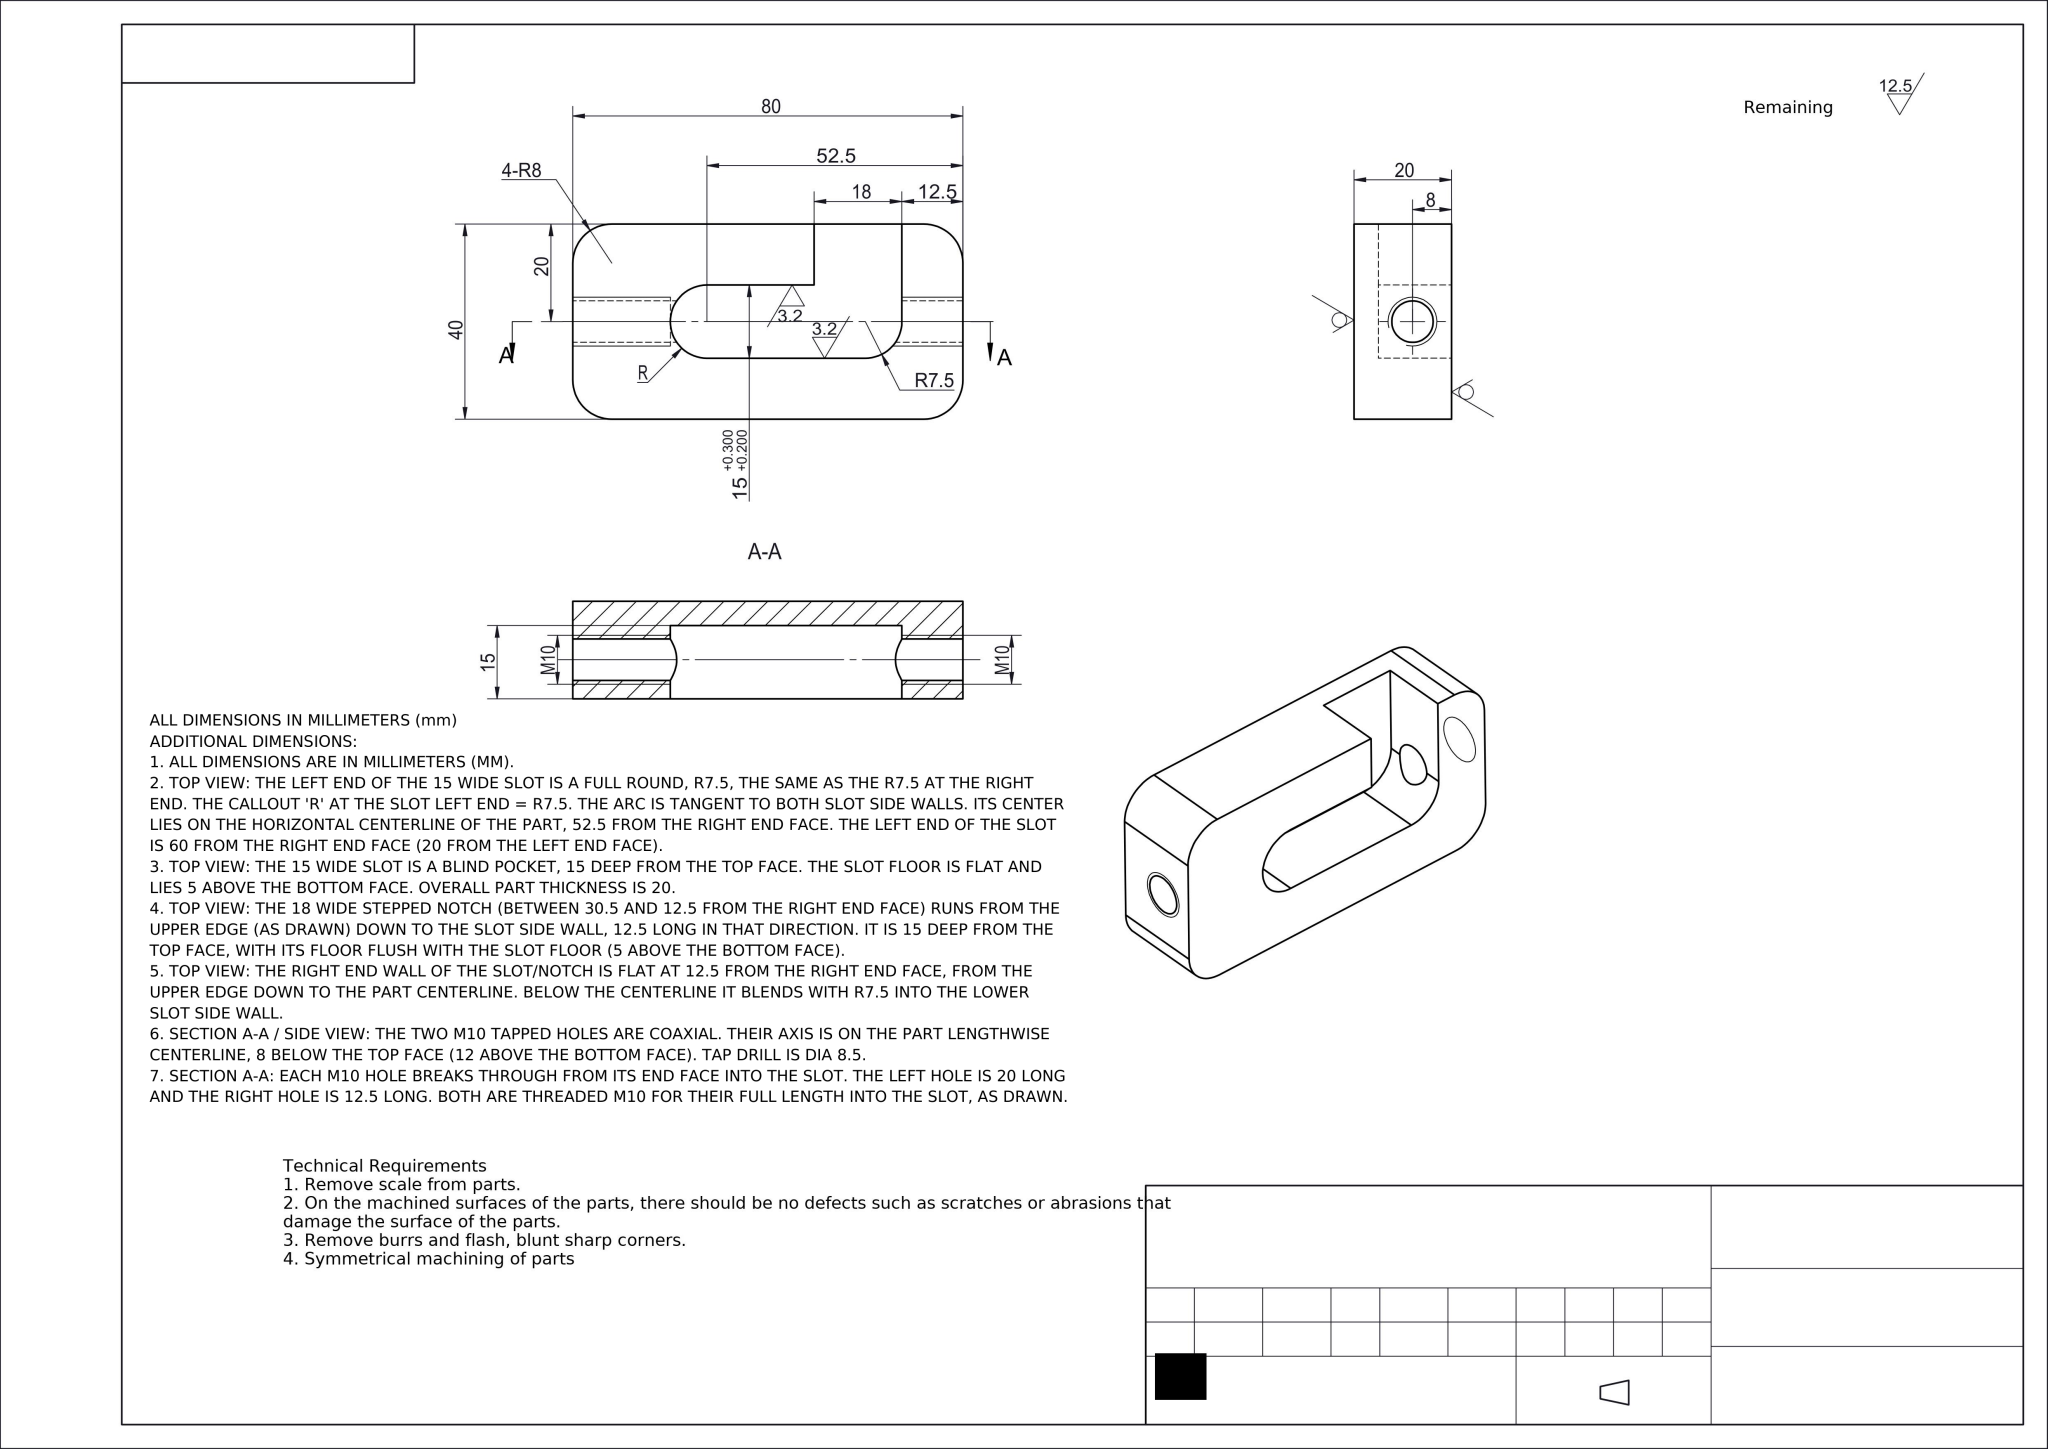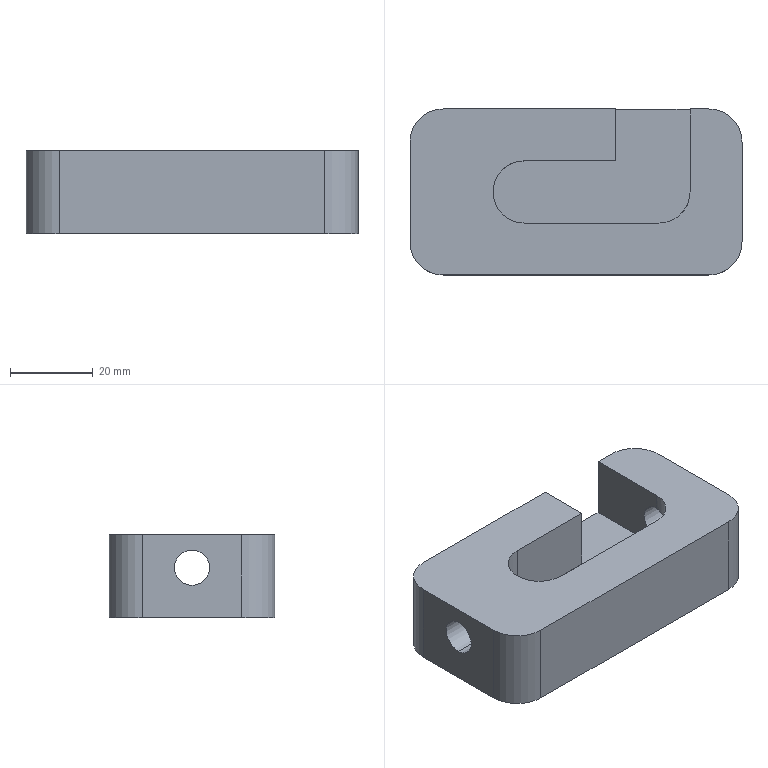Part | NX | mm | U-Shaped Slotted Clevis Bracket | 1 solid | 21 faces | box 80 x 40 x 20 mm | volume 47511 mm3 | plane 11 | cylinder 10 | commonest cylinder face diameters 8.5 x4 16 x4 15 x2
STEP:
#1=COLOUR_RGB('',1.,1.,1.);
#2=FILL_AREA_STYLE_COLOUR('',#1);
#3=FILL_AREA_STYLE('',(#2));
#4=SURFACE_STYLE_FILL_AREA(#3);
#5=SURFACE_SIDE_STYLE('',(#4));
#6=SURFACE_STYLE_USAGE(.BOTH.,#5);
#7=PRESENTATION_STYLE_ASSIGNMENT((#6));
#8=CARTESIAN_POINT('',(27.5,0.,16.25));
#9=VERTEX_POINT('',#8);
#10=CARTESIAN_POINT('',(27.5,0.,7.75));
#11=VERTEX_POINT('',#10);
#12=CARTESIAN_POINT('',(27.5,0.,16.25));
#13=CARTESIAN_POINT('',(27.5,-0.2876,16.25));
#14=CARTESIAN_POINT('',(27.484,-0.5693,16.221));
#15=CARTESIAN_POINT('',(27.421,-1.122,16.109));
#16=CARTESIAN_POINT('',(27.374,-1.395,16.024));
#17=CARTESIAN_POINT('',(27.258,-1.908,15.808));
#18=CARTESIAN_POINT('',(27.189,-2.15,15.676));
#19=CARTESIAN_POINT('',(27.036,-2.607,15.367));
#20=CARTESIAN_POINT('',(26.954,-2.818,15.193));
#21=CARTESIAN_POINT('',(26.786,-3.201,14.809));
#22=CARTESIAN_POINT('',(26.7,-3.376,14.597));
#23=CARTESIAN_POINT('',(26.537,-3.68,14.143));
#24=CARTESIAN_POINT('',(26.462,-3.81,13.904));
#25=CARTESIAN_POINT('',(26.331,-4.024,13.396));
#26=CARTESIAN_POINT('',(26.275,-4.108,13.124));
#27=CARTESIAN_POINT('',(26.2,-4.221,12.571));
#28=CARTESIAN_POINT('',(26.18,-4.25,12.289));
#29=CARTESIAN_POINT('',(26.18,-4.25,11.714));
#30=CARTESIAN_POINT('',(26.2,-4.221,11.432));
#31=CARTESIAN_POINT('',(26.274,-4.109,10.879));
#32=CARTESIAN_POINT('',(26.33,-4.025,10.607));
#33=CARTESIAN_POINT('',(26.461,-3.81,10.097));
#34=CARTESIAN_POINT('',(26.538,-3.678,9.854));
#35=CARTESIAN_POINT('',(26.701,-3.372,9.399));
#36=CARTESIAN_POINT('',(26.786,-3.2,9.19));
#37=CARTESIAN_POINT('',(26.955,-2.816,8.805));
#38=CARTESIAN_POINT('',(27.038,-2.602,8.628));
#39=CARTESIAN_POINT('',(27.19,-2.149,8.323));
#40=CARTESIAN_POINT('',(27.258,-1.908,8.192));
#41=CARTESIAN_POINT('',(27.345,-1.522,8.029));
#42=CARTESIAN_POINT('',(27.372,-1.389,7.981));
#43=CARTESIAN_POINT('',(27.417,-1.119,7.898));
#44=CARTESIAN_POINT('',(27.437,-0.9829,7.863));
#45=CARTESIAN_POINT('',(27.483,-0.5695,7.779));
#46=CARTESIAN_POINT('',(27.5,-0.288,7.75));
#47=CARTESIAN_POINT('',(27.5,0.,7.75));
#48=B_SPLINE_CURVE_WITH_KNOTS('',3,(#12,#13,#14,#15,#16,#17,#18,#19,#20,#21,#22,#23,#24,#25,#26,#27,#28,#29,#30,#31,#32,#33,#34,#35,#36,#37,#38,#39,#40,#41,#42,#43,#44,#45,#46,#47),.UNSPECIFIED.,.F.,.F.,(4,2,2,2,2,2,2,2,2,2,2,2,2,2,2,2,2,4),(0.,0.0008494,0.001699,0.002548,0.003398,0.004247,0.005097,0.005946,0.006796,0.007645,0.008494,0.009344,0.01019,0.01104,0.01189,0.01232,0.01274,0.01359),.UNSPECIFIED.);
#49=EDGE_CURVE('',#9,#11,#48,.T.);
#50=ORIENTED_EDGE('',*,*,#49,.F.);
#51=CARTESIAN_POINT('',(40.,-0.,16.25));
#52=VERTEX_POINT('',#51);
#53=CARTESIAN_POINT('',(40.,-0.,16.25));
#54=DIRECTION('',(1.,-0.,0.));
#55=VECTOR('',#54,1000.);
#56=LINE('',#53,#55);
#57=EDGE_CURVE('',#9,#52,#56,.T.);
#58=ORIENTED_EDGE('',*,*,#57,.T.);
#59=CARTESIAN_POINT('',(40.,-0.,7.75));
#60=VERTEX_POINT('',#59);
#61=CARTESIAN_POINT('',(40.,-0.,12.));
#62=DIRECTION('',(1.,-0.,0.));
#63=DIRECTION('',(0.,0.,-1.));
#64=AXIS2_PLACEMENT_3D('',#61,#62,#63);
#65=CIRCLE('',#64,4.25);
#66=EDGE_CURVE('',#52,#60,#65,.T.);
#67=ORIENTED_EDGE('',*,*,#66,.T.);
#68=CARTESIAN_POINT('',(40.,-0.,7.75));
#69=DIRECTION('',(1.,-0.,0.));
#70=VECTOR('',#69,1000.);
#71=LINE('',#68,#70);
#72=EDGE_CURVE('',#11,#60,#71,.T.);
#73=ORIENTED_EDGE('',*,*,#72,.F.);
#74=EDGE_LOOP('',(#50,#58,#67,#73));
#75=FACE_OUTER_BOUND('',#74,.T.);
#76=CARTESIAN_POINT('',(40.,-0.,12.));
#77=DIRECTION('',(1.,-0.,0.));
#78=DIRECTION('',(0.,0.,-1.));
#79=AXIS2_PLACEMENT_3D('',#76,#77,#78);
#80=CYLINDRICAL_SURFACE('',#79,4.25);
#81=ADVANCED_FACE('',(#75),#80,.F.);
#82=CARTESIAN_POINT('',(-20.,0.,7.75));
#83=VERTEX_POINT('',#82);
#84=CARTESIAN_POINT('',(-20.,0.,16.25));
#85=VERTEX_POINT('',#84);
#86=CARTESIAN_POINT('',(-20.,0.,7.75));
#87=CARTESIAN_POINT('',(-20.,-0.2872,7.75));
#88=CARTESIAN_POINT('',(-19.984,-0.5694,7.779));
#89=CARTESIAN_POINT('',(-19.921,-1.122,7.891));
#90=CARTESIAN_POINT('',(-19.874,-1.395,7.976));
#91=CARTESIAN_POINT('',(-19.758,-1.908,8.192));
#92=CARTESIAN_POINT('',(-19.689,-2.15,8.324));
#93=CARTESIAN_POINT('',(-19.536,-2.608,8.633));
#94=CARTESIAN_POINT('',(-19.454,-2.818,8.807));
#95=CARTESIAN_POINT('',(-19.286,-3.201,9.191));
#96=CARTESIAN_POINT('',(-19.2,-3.375,9.403));
#97=CARTESIAN_POINT('',(-19.038,-3.679,9.856));
#98=CARTESIAN_POINT('',(-18.962,-3.809,10.095));
#99=CARTESIAN_POINT('',(-18.831,-4.023,10.603));
#100=CARTESIAN_POINT('',(-18.775,-4.108,10.875));
#101=CARTESIAN_POINT('',(-18.7,-4.221,11.426));
#102=CARTESIAN_POINT('',(-18.68,-4.25,11.71));
#103=CARTESIAN_POINT('',(-18.679,-4.25,12.284));
#104=CARTESIAN_POINT('',(-18.699,-4.222,12.565));
#105=CARTESIAN_POINT('',(-18.774,-4.11,13.118));
#106=CARTESIAN_POINT('',(-18.829,-4.026,13.39));
#107=CARTESIAN_POINT('',(-18.96,-3.812,13.9));
#108=CARTESIAN_POINT('',(-19.038,-3.68,14.144));
#109=CARTESIAN_POINT('',(-19.2,-3.374,14.598));
#110=CARTESIAN_POINT('',(-19.285,-3.202,14.807));
#111=CARTESIAN_POINT('',(-19.453,-2.818,15.193));
#112=CARTESIAN_POINT('',(-19.537,-2.605,15.369));
#113=CARTESIAN_POINT('',(-19.688,-2.153,15.674));
#114=CARTESIAN_POINT('',(-19.757,-1.912,15.806));
#115=CARTESIAN_POINT('',(-19.873,-1.398,16.023));
#116=CARTESIAN_POINT('',(-19.92,-1.126,16.108));
#117=CARTESIAN_POINT('',(-19.983,-0.5735,16.221));
#118=CARTESIAN_POINT('',(-20.,-0.287,16.25));
#119=CARTESIAN_POINT('',(-20.,0.,16.25));
#120=B_SPLINE_CURVE_WITH_KNOTS('',3,(#86,#87,#88,#89,#90,#91,#92,#93,#94,#95,#96,#97,#98,#99,#100,#101,#102,#103,#104,#105,#106,#107,#108,#109,#110,#111,#112,#113,#114,#115,#116,#117,#118,#119),.UNSPECIFIED.,.F.,.F.,(4,2,2,2,2,2,2,2,2,2,2,2,2,2,2,2,4),(0.01359,0.01444,0.01529,0.01613,0.01698,0.01783,0.01868,0.01953,0.02037,0.02122,0.02207,0.02292,0.02376,0.02461,0.02546,0.02631,0.02716),.UNSPECIFIED.);
#121=EDGE_CURVE('',#83,#85,#120,.T.);
#122=ORIENTED_EDGE('',*,*,#121,.F.);
#123=CARTESIAN_POINT('',(-40.,0.,7.75));
#124=VERTEX_POINT('',#123);
#125=CARTESIAN_POINT('',(-40.,0.,7.75));
#126=DIRECTION('',(-1.,0.,-0.));
#127=VECTOR('',#126,1000.);
#128=LINE('',#125,#127);
#129=EDGE_CURVE('',#83,#124,#128,.T.);
#130=ORIENTED_EDGE('',*,*,#129,.T.);
#131=CARTESIAN_POINT('',(-40.,0.,16.25));
#132=VERTEX_POINT('',#131);
#133=CARTESIAN_POINT('',(-40.,0.,12.));
#134=DIRECTION('',(-1.,0.,-0.));
#135=DIRECTION('',(0.,0.,1.));
#136=AXIS2_PLACEMENT_3D('',#133,#134,#135);
#137=CIRCLE('',#136,4.25);
#138=EDGE_CURVE('',#124,#132,#137,.T.);
#139=ORIENTED_EDGE('',*,*,#138,.T.);
#140=CARTESIAN_POINT('',(-40.,0.,16.25));
#141=DIRECTION('',(-1.,0.,-0.));
#142=VECTOR('',#141,1000.);
#143=LINE('',#140,#142);
#144=EDGE_CURVE('',#85,#132,#143,.T.);
#145=ORIENTED_EDGE('',*,*,#144,.F.);
#146=EDGE_LOOP('',(#122,#130,#139,#145));
#147=FACE_OUTER_BOUND('',#146,.T.);
#148=CARTESIAN_POINT('',(-40.,0.,12.));
#149=DIRECTION('',(-1.,0.,-0.));
#150=DIRECTION('',(0.,0.,1.));
#151=AXIS2_PLACEMENT_3D('',#148,#149,#150);
#152=CYLINDRICAL_SURFACE('',#151,4.25);
#153=ADVANCED_FACE('',(#147),#152,.F.);
#154=CARTESIAN_POINT('',(-20.,0.,16.25));
#155=CARTESIAN_POINT('',(-20.,0.2876,16.25));
#156=CARTESIAN_POINT('',(-19.984,0.5693,16.221));
#157=CARTESIAN_POINT('',(-19.921,1.122,16.109));
#158=CARTESIAN_POINT('',(-19.874,1.395,16.024));
#159=CARTESIAN_POINT('',(-19.758,1.908,15.808));
#160=CARTESIAN_POINT('',(-19.689,2.15,15.676));
#161=CARTESIAN_POINT('',(-19.536,2.608,15.367));
#162=CARTESIAN_POINT('',(-19.454,2.818,15.193));
#163=CARTESIAN_POINT('',(-19.286,3.201,14.809));
#164=CARTESIAN_POINT('',(-19.2,3.376,14.596));
#165=CARTESIAN_POINT('',(-19.037,3.68,14.143));
#166=CARTESIAN_POINT('',(-18.961,3.81,13.903));
#167=CARTESIAN_POINT('',(-18.83,4.024,13.396));
#168=CARTESIAN_POINT('',(-18.775,4.108,13.124));
#169=CARTESIAN_POINT('',(-18.7,4.221,12.571));
#170=CARTESIAN_POINT('',(-18.68,4.25,12.289));
#171=CARTESIAN_POINT('',(-18.68,4.25,11.713));
#172=CARTESIAN_POINT('',(-18.7,4.221,11.432));
#173=CARTESIAN_POINT('',(-18.774,4.109,10.879));
#174=CARTESIAN_POINT('',(-18.83,4.025,10.607));
#175=CARTESIAN_POINT('',(-18.961,3.81,10.097));
#176=CARTESIAN_POINT('',(-19.038,3.678,9.853));
#177=CARTESIAN_POINT('',(-19.202,3.372,9.398));
#178=CARTESIAN_POINT('',(-19.287,3.199,9.189));
#179=CARTESIAN_POINT('',(-19.455,2.815,8.805));
#180=CARTESIAN_POINT('',(-19.538,2.602,8.628));
#181=CARTESIAN_POINT('',(-19.69,2.148,8.323));
#182=CARTESIAN_POINT('',(-19.758,1.907,8.192));
#183=CARTESIAN_POINT('',(-19.845,1.522,8.029));
#184=CARTESIAN_POINT('',(-19.872,1.388,7.981));
#185=CARTESIAN_POINT('',(-19.917,1.119,7.897));
#186=CARTESIAN_POINT('',(-19.937,0.9824,7.863));
#187=CARTESIAN_POINT('',(-19.984,0.5692,7.779));
#188=CARTESIAN_POINT('',(-20.,0.2878,7.75));
#189=CARTESIAN_POINT('',(-20.,0.,7.75));
#190=B_SPLINE_CURVE_WITH_KNOTS('',3,(#154,#155,#156,#157,#158,#159,#160,#161,#162,#163,#164,#165,#166,#167,#168,#169,#170,#171,#172,#173,#174,#175,#176,#177,#178,#179,#180,#181,#182,#183,#184,#185,#186,#187,#188,#189),.UNSPECIFIED.,.F.,.F.,(4,2,2,2,2,2,2,2,2,2,2,2,2,2,2,2,2,4),(0.,0.0008495,0.001699,0.002548,0.003398,0.004247,0.005097,0.005946,0.006796,0.007645,0.008495,0.009344,0.01019,0.01104,0.01189,0.01232,0.01274,0.01359),.UNSPECIFIED.);
#191=EDGE_CURVE('',#85,#83,#190,.T.);
#192=ORIENTED_EDGE('',*,*,#191,.T.);
#193=ORIENTED_EDGE('',*,*,#121,.T.);
#194=EDGE_LOOP('',(#192,#193));
#195=FACE_BOUND('',#194,.T.);
#196=CARTESIAN_POINT('',(-12.5,7.5,20.));
#197=VERTEX_POINT('',#196);
#198=CARTESIAN_POINT('',(-12.5,7.5,5.));
#199=VERTEX_POINT('',#198);
#200=CARTESIAN_POINT('',(-12.5,7.5,20.));
#201=DIRECTION('',(-0.,-0.,-1.));
#202=VECTOR('',#201,1000.);
#203=LINE('',#200,#202);
#204=EDGE_CURVE('',#197,#199,#203,.T.);
#205=ORIENTED_EDGE('',*,*,#204,.F.);
#206=CARTESIAN_POINT('',(-12.5,-7.5,20.));
#207=VERTEX_POINT('',#206);
#208=CARTESIAN_POINT('',(-12.5,-0.,20.));
#209=DIRECTION('',(0.,0.,1.));
#210=DIRECTION('',(1.,-0.,0.));
#211=AXIS2_PLACEMENT_3D('',#208,#209,#210);
#212=CIRCLE('',#211,7.5);
#213=EDGE_CURVE('',#197,#207,#212,.T.);
#214=ORIENTED_EDGE('',*,*,#213,.T.);
#215=CARTESIAN_POINT('',(-12.5,-7.5,5.));
#216=VERTEX_POINT('',#215);
#217=CARTESIAN_POINT('',(-12.5,-7.5,20.));
#218=DIRECTION('',(0.,0.,1.));
#219=VECTOR('',#218,1000.);
#220=LINE('',#217,#219);
#221=EDGE_CURVE('',#216,#207,#220,.T.);
#222=ORIENTED_EDGE('',*,*,#221,.F.);
#223=CARTESIAN_POINT('',(-12.5,0.,5.));
#224=DIRECTION('',(0.,0.,1.));
#225=DIRECTION('',(1.,-0.,0.));
#226=AXIS2_PLACEMENT_3D('',#223,#224,#225);
#227=CIRCLE('',#226,7.5);
#228=EDGE_CURVE('',#199,#216,#227,.T.);
#229=ORIENTED_EDGE('',*,*,#228,.F.);
#230=EDGE_LOOP('',(#205,#214,#222,#229));
#231=FACE_OUTER_BOUND('',#230,.T.);
#232=CARTESIAN_POINT('',(-12.5,-0.,20.));
#233=DIRECTION('',(0.,0.,1.));
#234=DIRECTION('',(1.,-0.,0.));
#235=AXIS2_PLACEMENT_3D('',#232,#233,#234);
#236=CYLINDRICAL_SURFACE('',#235,7.5);
#237=ADVANCED_FACE('',(#195,#231),#236,.F.);
#238=CARTESIAN_POINT('',(40.,-0.,12.));
#239=DIRECTION('',(1.,-0.,0.));
#240=DIRECTION('',(0.,0.,-1.));
#241=AXIS2_PLACEMENT_3D('',#238,#239,#240);
#242=CIRCLE('',#241,4.25);
#243=EDGE_CURVE('',#60,#52,#242,.T.);
#244=ORIENTED_EDGE('',*,*,#243,.F.);
#245=ORIENTED_EDGE('',*,*,#66,.F.);
#246=EDGE_LOOP('',(#244,#245));
#247=FACE_BOUND('',#246,.T.);
#248=CARTESIAN_POINT('',(40.,-12.,20.));
#249=VERTEX_POINT('',#248);
#250=CARTESIAN_POINT('',(40.,12.,20.));
#251=VERTEX_POINT('',#250);
#252=CARTESIAN_POINT('',(40.,20.,20.));
#253=DIRECTION('',(-0.,1.,0.));
#254=VECTOR('',#253,1000.);
#255=LINE('',#252,#254);
#256=EDGE_CURVE('',#249,#251,#255,.T.);
#257=ORIENTED_EDGE('',*,*,#256,.F.);
#258=CARTESIAN_POINT('',(40.,-12.,0.));
#259=VERTEX_POINT('',#258);
#260=CARTESIAN_POINT('',(40.,-12.,20.));
#261=DIRECTION('',(-0.,-0.,-1.));
#262=VECTOR('',#261,1000.);
#263=LINE('',#260,#262);
#264=EDGE_CURVE('',#249,#259,#263,.T.);
#265=ORIENTED_EDGE('',*,*,#264,.T.);
#266=CARTESIAN_POINT('',(40.,12.,0.));
#267=VERTEX_POINT('',#266);
#268=CARTESIAN_POINT('',(40.,20.,0.));
#269=DIRECTION('',(-0.,1.,0.));
#270=VECTOR('',#269,1000.);
#271=LINE('',#268,#270);
#272=EDGE_CURVE('',#259,#267,#271,.T.);
#273=ORIENTED_EDGE('',*,*,#272,.T.);
#274=CARTESIAN_POINT('',(40.,12.,20.));
#275=DIRECTION('',(0.,0.,1.));
#276=VECTOR('',#275,1000.);
#277=LINE('',#274,#276);
#278=EDGE_CURVE('',#267,#251,#277,.T.);
#279=ORIENTED_EDGE('',*,*,#278,.T.);
#280=EDGE_LOOP('',(#257,#265,#273,#279));
#281=FACE_OUTER_BOUND('',#280,.T.);
#282=CARTESIAN_POINT('',(40.,20.,20.));
#283=DIRECTION('',(-1.,-0.,-0.));
#284=DIRECTION('',(0.,-1.,-0.));
#285=AXIS2_PLACEMENT_3D('',#282,#283,#284);
#286=PLANE('',#285);
#287=ADVANCED_FACE('',(#247,#281),#286,.F.);
#288=CARTESIAN_POINT('',(32.,20.,20.));
#289=VERTEX_POINT('',#288);
#290=CARTESIAN_POINT('',(27.5,20.,20.));
#291=VERTEX_POINT('',#290);
#292=CARTESIAN_POINT('',(-40.,20.,20.));
#293=DIRECTION('',(-1.,0.,-0.));
#294=VECTOR('',#293,1000.);
#295=LINE('',#292,#294);
#296=EDGE_CURVE('',#289,#291,#295,.T.);
#297=ORIENTED_EDGE('',*,*,#296,.F.);
#298=CARTESIAN_POINT('',(32.,20.,0.));
#299=VERTEX_POINT('',#298);
#300=CARTESIAN_POINT('',(32.,20.,20.));
#301=DIRECTION('',(-0.,-0.,-1.));
#302=VECTOR('',#301,1000.);
#303=LINE('',#300,#302);
#304=EDGE_CURVE('',#289,#299,#303,.T.);
#305=ORIENTED_EDGE('',*,*,#304,.T.);
#306=CARTESIAN_POINT('',(-32.,20.,0.));
#307=VERTEX_POINT('',#306);
#308=CARTESIAN_POINT('',(-40.,20.,0.));
#309=DIRECTION('',(-1.,0.,-0.));
#310=VECTOR('',#309,1000.);
#311=LINE('',#308,#310);
#312=EDGE_CURVE('',#299,#307,#311,.T.);
#313=ORIENTED_EDGE('',*,*,#312,.T.);
#314=CARTESIAN_POINT('',(-32.,20.,20.));
#315=VERTEX_POINT('',#314);
#316=CARTESIAN_POINT('',(-32.,20.,20.));
#317=DIRECTION('',(0.,0.,1.));
#318=VECTOR('',#317,1000.);
#319=LINE('',#316,#318);
#320=EDGE_CURVE('',#307,#315,#319,.T.);
#321=ORIENTED_EDGE('',*,*,#320,.T.);
#322=CARTESIAN_POINT('',(9.5,20.,20.));
#323=VERTEX_POINT('',#322);
#324=CARTESIAN_POINT('',(-40.,20.,20.));
#325=DIRECTION('',(-1.,0.,-0.));
#326=VECTOR('',#325,1000.);
#327=LINE('',#324,#326);
#328=EDGE_CURVE('',#323,#315,#327,.T.);
#329=ORIENTED_EDGE('',*,*,#328,.F.);
#330=CARTESIAN_POINT('',(9.5,20.,5.));
#331=VERTEX_POINT('',#330);
#332=CARTESIAN_POINT('',(9.5,20.,20.));
#333=DIRECTION('',(-0.,-0.,-1.));
#334=VECTOR('',#333,1000.);
#335=LINE('',#332,#334);
#336=EDGE_CURVE('',#323,#331,#335,.T.);
#337=ORIENTED_EDGE('',*,*,#336,.T.);
#338=CARTESIAN_POINT('',(27.5,20.,5.));
#339=VERTEX_POINT('',#338);
#340=CARTESIAN_POINT('',(-40.,20.,5.));
#341=DIRECTION('',(-1.,0.,-0.));
#342=VECTOR('',#341,1000.);
#343=LINE('',#340,#342);
#344=EDGE_CURVE('',#339,#331,#343,.T.);
#345=ORIENTED_EDGE('',*,*,#344,.F.);
#346=CARTESIAN_POINT('',(27.5,20.,20.));
#347=DIRECTION('',(0.,0.,1.));
#348=VECTOR('',#347,1000.);
#349=LINE('',#346,#348);
#350=EDGE_CURVE('',#339,#291,#349,.T.);
#351=ORIENTED_EDGE('',*,*,#350,.T.);
#352=EDGE_LOOP('',(#297,#305,#313,#321,#329,#337,#345,#351));
#353=FACE_OUTER_BOUND('',#352,.T.);
#354=CARTESIAN_POINT('',(-40.,20.,20.));
#355=DIRECTION('',(0.,-1.,0.));
#356=DIRECTION('',(-0.,-0.,-1.));
#357=AXIS2_PLACEMENT_3D('',#354,#355,#356);
#358=PLANE('',#357);
#359=ADVANCED_FACE('',(#353),#358,.F.);
#360=CARTESIAN_POINT('',(-40.,0.,12.));
#361=DIRECTION('',(-1.,0.,-0.));
#362=DIRECTION('',(0.,0.,1.));
#363=AXIS2_PLACEMENT_3D('',#360,#361,#362);
#364=CIRCLE('',#363,4.25);
#365=EDGE_CURVE('',#132,#124,#364,.T.);
#366=ORIENTED_EDGE('',*,*,#365,.F.);
#367=ORIENTED_EDGE('',*,*,#138,.F.);
#368=EDGE_LOOP('',(#366,#367));
#369=FACE_BOUND('',#368,.T.);
#370=CARTESIAN_POINT('',(-40.,12.,0.));
#371=VERTEX_POINT('',#370);
#372=CARTESIAN_POINT('',(-40.,-12.,0.));
#373=VERTEX_POINT('',#372);
#374=CARTESIAN_POINT('',(-40.,20.,0.));
#375=DIRECTION('',(0.,-1.,-0.));
#376=VECTOR('',#375,1000.);
#377=LINE('',#374,#376);
#378=EDGE_CURVE('',#371,#373,#377,.T.);
#379=ORIENTED_EDGE('',*,*,#378,.T.);
#380=CARTESIAN_POINT('',(-40.,-12.,20.));
#381=VERTEX_POINT('',#380);
#382=CARTESIAN_POINT('',(-40.,-12.,20.));
#383=DIRECTION('',(0.,0.,1.));
#384=VECTOR('',#383,1000.);
#385=LINE('',#382,#384);
#386=EDGE_CURVE('',#373,#381,#385,.T.);
#387=ORIENTED_EDGE('',*,*,#386,.T.);
#388=CARTESIAN_POINT('',(-40.,12.,20.));
#389=VERTEX_POINT('',#388);
#390=CARTESIAN_POINT('',(-40.,20.,20.));
#391=DIRECTION('',(0.,-1.,-0.));
#392=VECTOR('',#391,1000.);
#393=LINE('',#390,#392);
#394=EDGE_CURVE('',#389,#381,#393,.T.);
#395=ORIENTED_EDGE('',*,*,#394,.F.);
#396=CARTESIAN_POINT('',(-40.,12.,20.));
#397=DIRECTION('',(-0.,-0.,-1.));
#398=VECTOR('',#397,1000.);
#399=LINE('',#396,#398);
#400=EDGE_CURVE('',#389,#371,#399,.T.);
#401=ORIENTED_EDGE('',*,*,#400,.T.);
#402=EDGE_LOOP('',(#379,#387,#395,#401));
#403=FACE_OUTER_BOUND('',#402,.T.);
#404=CARTESIAN_POINT('',(-40.,20.,20.));
#405=DIRECTION('',(1.,0.,0.));
#406=DIRECTION('',(-0.,1.,0.));
#407=AXIS2_PLACEMENT_3D('',#404,#405,#406);
#408=PLANE('',#407);
#409=ADVANCED_FACE('',(#369,#403),#408,.F.);
#410=CARTESIAN_POINT('',(-32.,-20.,0.));
#411=VERTEX_POINT('',#410);
#412=CARTESIAN_POINT('',(32.,-20.,0.));
#413=VERTEX_POINT('',#412);
#414=CARTESIAN_POINT('',(-40.,-20.,0.));
#415=DIRECTION('',(1.,-0.,0.));
#416=VECTOR('',#415,1000.);
#417=LINE('',#414,#416);
#418=EDGE_CURVE('',#411,#413,#417,.T.);
#419=ORIENTED_EDGE('',*,*,#418,.T.);
#420=CARTESIAN_POINT('',(32.,-20.,20.));
#421=VERTEX_POINT('',#420);
#422=CARTESIAN_POINT('',(32.,-20.,20.));
#423=DIRECTION('',(0.,0.,1.));
#424=VECTOR('',#423,1000.);
#425=LINE('',#422,#424);
#426=EDGE_CURVE('',#413,#421,#425,.T.);
#427=ORIENTED_EDGE('',*,*,#426,.T.);
#428=CARTESIAN_POINT('',(-32.,-20.,20.));
#429=VERTEX_POINT('',#428);
#430=CARTESIAN_POINT('',(-40.,-20.,20.));
#431=DIRECTION('',(1.,-0.,0.));
#432=VECTOR('',#431,1000.);
#433=LINE('',#430,#432);
#434=EDGE_CURVE('',#429,#421,#433,.T.);
#435=ORIENTED_EDGE('',*,*,#434,.F.);
#436=CARTESIAN_POINT('',(-32.,-20.,20.));
#437=DIRECTION('',(-0.,-0.,-1.));
#438=VECTOR('',#437,1000.);
#439=LINE('',#436,#438);
#440=EDGE_CURVE('',#429,#411,#439,.T.);
#441=ORIENTED_EDGE('',*,*,#440,.T.);
#442=EDGE_LOOP('',(#419,#427,#435,#441));
#443=FACE_OUTER_BOUND('',#442,.T.);
#444=CARTESIAN_POINT('',(-40.,-20.,20.));
#445=DIRECTION('',(-0.,1.,-0.));
#446=DIRECTION('',(0.,0.,1.));
#447=AXIS2_PLACEMENT_3D('',#444,#445,#446);
#448=PLANE('',#447);
#449=ADVANCED_FACE('',(#443),#448,.F.);
#450=ORIENTED_EDGE('',*,*,#434,.T.);
#451=CARTESIAN_POINT('',(32.,-12.,20.));
#452=DIRECTION('',(0.,0.,1.));
#453=DIRECTION('',(1.,0.,0.));
#454=AXIS2_PLACEMENT_3D('',#451,#452,#453);
#455=CIRCLE('',#454,8.);
#456=EDGE_CURVE('',#421,#249,#455,.T.);
#457=ORIENTED_EDGE('',*,*,#456,.T.);
#458=ORIENTED_EDGE('',*,*,#256,.T.);
#459=CARTESIAN_POINT('',(32.,12.,20.));
#460=DIRECTION('',(0.,0.,1.));
#461=DIRECTION('',(1.,0.,0.));
#462=AXIS2_PLACEMENT_3D('',#459,#460,#461);
#463=CIRCLE('',#462,8.);
#464=EDGE_CURVE('',#251,#289,#463,.T.);
#465=ORIENTED_EDGE('',*,*,#464,.T.);
#466=ORIENTED_EDGE('',*,*,#296,.T.);
#467=CARTESIAN_POINT('',(27.5,0.,20.));
#468=VERTEX_POINT('',#467);
#469=CARTESIAN_POINT('',(27.5,7.5,20.));
#470=DIRECTION('',(-0.,1.,0.));
#471=VECTOR('',#470,1000.);
#472=LINE('',#469,#471);
#473=EDGE_CURVE('',#468,#291,#472,.T.);
#474=ORIENTED_EDGE('',*,*,#473,.F.);
#475=CARTESIAN_POINT('',(20.,-7.5,20.));
#476=VERTEX_POINT('',#475);
#477=CARTESIAN_POINT('',(20.,0.,20.));
#478=DIRECTION('',(-0.,-0.,-1.));
#479=DIRECTION('',(1.,-0.,0.));
#480=AXIS2_PLACEMENT_3D('',#477,#478,#479);
#481=CIRCLE('',#480,7.5);
#482=EDGE_CURVE('',#468,#476,#481,.T.);
#483=ORIENTED_EDGE('',*,*,#482,.T.);
#484=CARTESIAN_POINT('',(-20.,-7.5,20.));
#485=DIRECTION('',(1.,-0.,0.));
#486=VECTOR('',#485,1000.);
#487=LINE('',#484,#486);
#488=EDGE_CURVE('',#207,#476,#487,.T.);
#489=ORIENTED_EDGE('',*,*,#488,.F.);
#490=ORIENTED_EDGE('',*,*,#213,.F.);
#491=CARTESIAN_POINT('',(9.5,7.5,20.));
#492=VERTEX_POINT('',#491);
#493=CARTESIAN_POINT('',(-20.,7.5,20.));
#494=DIRECTION('',(-1.,0.,-0.));
#495=VECTOR('',#494,1000.);
#496=LINE('',#493,#495);
#497=EDGE_CURVE('',#492,#197,#496,.T.);
#498=ORIENTED_EDGE('',*,*,#497,.F.);
#499=CARTESIAN_POINT('',(9.5,47.125,20.));
#500=DIRECTION('',(0.,-1.,-0.));
#501=VECTOR('',#500,1000.);
#502=LINE('',#499,#501);
#503=EDGE_CURVE('',#323,#492,#502,.T.);
#504=ORIENTED_EDGE('',*,*,#503,.F.);
#505=ORIENTED_EDGE('',*,*,#328,.T.);
#506=CARTESIAN_POINT('',(-32.,12.,20.));
#507=DIRECTION('',(0.,0.,1.));
#508=DIRECTION('',(1.,0.,0.));
#509=AXIS2_PLACEMENT_3D('',#506,#507,#508);
#510=CIRCLE('',#509,8.);
#511=EDGE_CURVE('',#315,#389,#510,.T.);
#512=ORIENTED_EDGE('',*,*,#511,.T.);
#513=ORIENTED_EDGE('',*,*,#394,.T.);
#514=CARTESIAN_POINT('',(-32.,-12.,20.));
#515=DIRECTION('',(0.,0.,1.));
#516=DIRECTION('',(1.,0.,0.));
#517=AXIS2_PLACEMENT_3D('',#514,#515,#516);
#518=CIRCLE('',#517,8.);
#519=EDGE_CURVE('',#381,#429,#518,.T.);
#520=ORIENTED_EDGE('',*,*,#519,.T.);
#521=EDGE_LOOP('',(#450,#457,#458,#465,#466,#474,#483,#489,#490,#498,#504,#505,#512,#513,#520));
#522=FACE_OUTER_BOUND('',#521,.T.);
#523=CARTESIAN_POINT('',(0.,0.,20.));
#524=DIRECTION('',(-0.,0.,1.));
#525=DIRECTION('',(1.,-0.,0.));
#526=AXIS2_PLACEMENT_3D('',#523,#524,#525);
#527=PLANE('',#526);
#528=ADVANCED_FACE('',(#522),#527,.T.);
#529=ORIENTED_EDGE('',*,*,#272,.F.);
#530=CARTESIAN_POINT('',(32.,-12.,0.));
#531=DIRECTION('',(-0.,-0.,-1.));
#532=DIRECTION('',(1.,0.,0.));
#533=AXIS2_PLACEMENT_3D('',#530,#531,#532);
#534=CIRCLE('',#533,8.);
#535=EDGE_CURVE('',#259,#413,#534,.T.);
#536=ORIENTED_EDGE('',*,*,#535,.T.);
#537=ORIENTED_EDGE('',*,*,#418,.F.);
#538=CARTESIAN_POINT('',(-32.,-12.,0.));
#539=DIRECTION('',(-0.,-0.,-1.));
#540=DIRECTION('',(1.,0.,0.));
#541=AXIS2_PLACEMENT_3D('',#538,#539,#540);
#542=CIRCLE('',#541,8.);
#543=EDGE_CURVE('',#411,#373,#542,.T.);
#544=ORIENTED_EDGE('',*,*,#543,.T.);
#545=ORIENTED_EDGE('',*,*,#378,.F.);
#546=CARTESIAN_POINT('',(-32.,12.,0.));
#547=DIRECTION('',(-0.,-0.,-1.));
#548=DIRECTION('',(1.,0.,0.));
#549=AXIS2_PLACEMENT_3D('',#546,#547,#548);
#550=CIRCLE('',#549,8.);
#551=EDGE_CURVE('',#371,#307,#550,.T.);
#552=ORIENTED_EDGE('',*,*,#551,.T.);
#553=ORIENTED_EDGE('',*,*,#312,.F.);
#554=CARTESIAN_POINT('',(32.,12.,0.));
#555=DIRECTION('',(-0.,-0.,-1.));
#556=DIRECTION('',(1.,0.,0.));
#557=AXIS2_PLACEMENT_3D('',#554,#555,#556);
#558=CIRCLE('',#557,8.);
#559=EDGE_CURVE('',#299,#267,#558,.T.);
#560=ORIENTED_EDGE('',*,*,#559,.T.);
#561=EDGE_LOOP('',(#529,#536,#537,#544,#545,#552,#553,#560));
#562=FACE_OUTER_BOUND('',#561,.T.);
#563=CARTESIAN_POINT('',(0.,0.,0.));
#564=DIRECTION('',(-0.,0.,1.));
#565=DIRECTION('',(1.,-0.,0.));
#566=AXIS2_PLACEMENT_3D('',#563,#564,#565);
#567=PLANE('',#566);
#568=ADVANCED_FACE('',(#562),#567,.F.);
#569=CARTESIAN_POINT('',(27.5,0.,5.));
#570=VERTEX_POINT('',#569);
#571=CARTESIAN_POINT('',(27.5,0.,20.));
#572=DIRECTION('',(0.,0.,1.));
#573=VECTOR('',#572,1000.);
#574=LINE('',#571,#573);
#575=EDGE_CURVE('',#570,#11,#574,.T.);
#576=ORIENTED_EDGE('',*,*,#575,.T.);
#577=CARTESIAN_POINT('',(27.5,0.,12.));
#578=DIRECTION('',(1.,0.,0.));
#579=DIRECTION('',(-0.,1.,0.));
#580=AXIS2_PLACEMENT_3D('',#577,#578,#579);
#581=CIRCLE('',#580,4.25);
#582=EDGE_CURVE('',#11,#9,#581,.T.);
#583=ORIENTED_EDGE('',*,*,#582,.T.);
#584=CARTESIAN_POINT('',(27.5,0.,20.));
#585=DIRECTION('',(0.,0.,1.));
#586=VECTOR('',#585,1000.);
#587=LINE('',#584,#586);
#588=EDGE_CURVE('',#9,#468,#587,.T.);
#589=ORIENTED_EDGE('',*,*,#588,.T.);
#590=ORIENTED_EDGE('',*,*,#473,.T.);
#591=ORIENTED_EDGE('',*,*,#350,.F.);
#592=CARTESIAN_POINT('',(27.5,7.5,5.));
#593=DIRECTION('',(-0.,1.,0.));
#594=VECTOR('',#593,1000.);
#595=LINE('',#592,#594);
#596=EDGE_CURVE('',#570,#339,#595,.T.);
#597=ORIENTED_EDGE('',*,*,#596,.F.);
#598=EDGE_LOOP('',(#576,#583,#589,#590,#591,#597));
#599=FACE_OUTER_BOUND('',#598,.T.);
#600=CARTESIAN_POINT('',(27.5,7.5,5.));
#601=DIRECTION('',(1.,0.,0.));
#602=DIRECTION('',(-0.,1.,0.));
#603=AXIS2_PLACEMENT_3D('',#600,#601,#602);
#604=PLANE('',#603);
#605=ADVANCED_FACE('',(#599),#604,.F.);
#606=ORIENTED_EDGE('',*,*,#488,.T.);
#607=CARTESIAN_POINT('',(20.,-7.5,5.));
#608=VERTEX_POINT('',#607);
#609=CARTESIAN_POINT('',(20.,-7.5,5.));
#610=DIRECTION('',(-0.,-0.,-1.));
#611=VECTOR('',#610,1000.);
#612=LINE('',#609,#611);
#613=EDGE_CURVE('',#476,#608,#612,.T.);
#614=ORIENTED_EDGE('',*,*,#613,.T.);
#615=CARTESIAN_POINT('',(-20.,-7.5,5.));
#616=DIRECTION('',(1.,-0.,0.));
#617=VECTOR('',#616,1000.);
#618=LINE('',#615,#617);
#619=EDGE_CURVE('',#216,#608,#618,.T.);
#620=ORIENTED_EDGE('',*,*,#619,.F.);
#621=ORIENTED_EDGE('',*,*,#221,.T.);
#622=EDGE_LOOP('',(#606,#614,#620,#621));
#623=FACE_OUTER_BOUND('',#622,.T.);
#624=CARTESIAN_POINT('',(-20.,-7.5,5.));
#625=DIRECTION('',(-0.,-1.,-0.));
#626=DIRECTION('',(1.,-0.,0.));
#627=AXIS2_PLACEMENT_3D('',#624,#625,#626);
#628=PLANE('',#627);
#629=ADVANCED_FACE('',(#623),#628,.F.);
#630=CARTESIAN_POINT('',(9.5,7.5,5.));
#631=VERTEX_POINT('',#630);
#632=CARTESIAN_POINT('',(-20.,7.5,5.));
#633=DIRECTION('',(-1.,0.,-0.));
#634=VECTOR('',#633,1000.);
#635=LINE('',#632,#634);
#636=EDGE_CURVE('',#631,#199,#635,.T.);
#637=ORIENTED_EDGE('',*,*,#636,.F.);
#638=CARTESIAN_POINT('',(9.5,7.5,5.));
#639=DIRECTION('',(0.,0.,1.));
#640=VECTOR('',#639,1000.);
#641=LINE('',#638,#640);
#642=EDGE_CURVE('',#631,#492,#641,.T.);
#643=ORIENTED_EDGE('',*,*,#642,.T.);
#644=ORIENTED_EDGE('',*,*,#497,.T.);
#645=ORIENTED_EDGE('',*,*,#204,.T.);
#646=EDGE_LOOP('',(#637,#643,#644,#645));
#647=FACE_OUTER_BOUND('',#646,.T.);
#648=CARTESIAN_POINT('',(-20.,7.5,5.));
#649=DIRECTION('',(-0.,1.,-0.));
#650=DIRECTION('',(0.,0.,1.));
#651=AXIS2_PLACEMENT_3D('',#648,#649,#650);
#652=PLANE('',#651);
#653=ADVANCED_FACE('',(#647),#652,.F.);
#654=ORIENTED_EDGE('',*,*,#619,.T.);
#655=CARTESIAN_POINT('',(20.,0.,5.));
#656=DIRECTION('',(0.,0.,1.));
#657=DIRECTION('',(1.,-0.,0.));
#658=AXIS2_PLACEMENT_3D('',#655,#656,#657);
#659=CIRCLE('',#658,7.5);
#660=EDGE_CURVE('',#608,#570,#659,.T.);
#661=ORIENTED_EDGE('',*,*,#660,.T.);
#662=ORIENTED_EDGE('',*,*,#596,.T.);
#663=ORIENTED_EDGE('',*,*,#344,.T.);
#664=CARTESIAN_POINT('',(9.5,47.125,5.));
#665=DIRECTION('',(0.,-1.,-0.));
#666=VECTOR('',#665,1000.);
#667=LINE('',#664,#666);
#668=EDGE_CURVE('',#331,#631,#667,.T.);
#669=ORIENTED_EDGE('',*,*,#668,.T.);
#670=ORIENTED_EDGE('',*,*,#636,.T.);
#671=ORIENTED_EDGE('',*,*,#228,.T.);
#672=EDGE_LOOP('',(#654,#661,#662,#663,#669,#670,#671));
#673=FACE_OUTER_BOUND('',#672,.T.);
#674=CARTESIAN_POINT('',(0.,0.,5.));
#675=DIRECTION('',(-0.,0.,1.));
#676=DIRECTION('',(1.,-0.,0.));
#677=AXIS2_PLACEMENT_3D('',#674,#675,#676);
#678=PLANE('',#677);
#679=ADVANCED_FACE('',(#673),#678,.T.);
#680=ORIENTED_EDGE('',*,*,#503,.T.);
#681=ORIENTED_EDGE('',*,*,#642,.F.);
#682=ORIENTED_EDGE('',*,*,#668,.F.);
#683=ORIENTED_EDGE('',*,*,#336,.F.);
#684=EDGE_LOOP('',(#680,#681,#682,#683));
#685=FACE_OUTER_BOUND('',#684,.T.);
#686=CARTESIAN_POINT('',(9.5,47.125,5.));
#687=DIRECTION('',(-1.,-0.,-0.));
#688=DIRECTION('',(0.,-1.,-0.));
#689=AXIS2_PLACEMENT_3D('',#686,#687,#688);
#690=PLANE('',#689);
#691=ADVANCED_FACE('',(#685),#690,.F.);
#692=ORIENTED_EDGE('',*,*,#588,.F.);
#693=ORIENTED_EDGE('',*,*,#49,.T.);
#694=ORIENTED_EDGE('',*,*,#575,.F.);
#695=ORIENTED_EDGE('',*,*,#660,.F.);
#696=ORIENTED_EDGE('',*,*,#613,.F.);
#697=ORIENTED_EDGE('',*,*,#482,.F.);
#698=EDGE_LOOP('',(#692,#693,#694,#695,#696,#697));
#699=FACE_OUTER_BOUND('',#698,.T.);
#700=CARTESIAN_POINT('',(20.,0.,5.));
#701=DIRECTION('',(-0.,-0.,-1.));
#702=DIRECTION('',(-1.,0.,0.));
#703=AXIS2_PLACEMENT_3D('',#700,#701,#702);
#704=CYLINDRICAL_SURFACE('',#703,7.5);
#705=ADVANCED_FACE('',(#699),#704,.F.);
#706=ORIENTED_EDGE('',*,*,#129,.F.);
#707=ORIENTED_EDGE('',*,*,#191,.F.);
#708=ORIENTED_EDGE('',*,*,#144,.T.);
#709=ORIENTED_EDGE('',*,*,#365,.T.);
#710=EDGE_LOOP('',(#706,#707,#708,#709));
#711=FACE_OUTER_BOUND('',#710,.T.);
#712=CARTESIAN_POINT('',(-40.,0.,12.));
#713=DIRECTION('',(-1.,0.,-0.));
#714=DIRECTION('',(0.,0.,1.));
#715=AXIS2_PLACEMENT_3D('',#712,#713,#714);
#716=CYLINDRICAL_SURFACE('',#715,4.25);
#717=ADVANCED_FACE('',(#711),#716,.F.);
#718=ORIENTED_EDGE('',*,*,#57,.F.);
#719=ORIENTED_EDGE('',*,*,#582,.F.);
#720=ORIENTED_EDGE('',*,*,#72,.T.);
#721=ORIENTED_EDGE('',*,*,#243,.T.);
#722=EDGE_LOOP('',(#718,#719,#720,#721));
#723=FACE_OUTER_BOUND('',#722,.T.);
#724=CARTESIAN_POINT('',(40.,-0.,12.));
#725=DIRECTION('',(1.,-0.,0.));
#726=DIRECTION('',(0.,0.,-1.));
#727=AXIS2_PLACEMENT_3D('',#724,#725,#726);
#728=CYLINDRICAL_SURFACE('',#727,4.25);
#729=ADVANCED_FACE('',(#723),#728,.F.);
#730=ORIENTED_EDGE('',*,*,#456,.F.);
#731=ORIENTED_EDGE('',*,*,#426,.F.);
#732=ORIENTED_EDGE('',*,*,#535,.F.);
#733=ORIENTED_EDGE('',*,*,#264,.F.);
#734=EDGE_LOOP('',(#730,#731,#732,#733));
#735=FACE_OUTER_BOUND('',#734,.T.);
#736=CARTESIAN_POINT('',(32.,-12.,20.));
#737=DIRECTION('',(-0.,-0.,-1.));
#738=DIRECTION('',(-1.,0.,0.));
#739=AXIS2_PLACEMENT_3D('',#736,#737,#738);
#740=CYLINDRICAL_SURFACE('',#739,8.);
#741=ADVANCED_FACE('',(#735),#740,.T.);
#742=ORIENTED_EDGE('',*,*,#464,.F.);
#743=ORIENTED_EDGE('',*,*,#278,.F.);
#744=ORIENTED_EDGE('',*,*,#559,.F.);
#745=ORIENTED_EDGE('',*,*,#304,.F.);
#746=EDGE_LOOP('',(#742,#743,#744,#745));
#747=FACE_OUTER_BOUND('',#746,.T.);
#748=CARTESIAN_POINT('',(32.,12.,20.));
#749=DIRECTION('',(-0.,-0.,-1.));
#750=DIRECTION('',(-1.,0.,0.));
#751=AXIS2_PLACEMENT_3D('',#748,#749,#750);
#752=CYLINDRICAL_SURFACE('',#751,8.);
#753=ADVANCED_FACE('',(#747),#752,.T.);
#754=ORIENTED_EDGE('',*,*,#519,.F.);
#755=ORIENTED_EDGE('',*,*,#386,.F.);
#756=ORIENTED_EDGE('',*,*,#543,.F.);
#757=ORIENTED_EDGE('',*,*,#440,.F.);
#758=EDGE_LOOP('',(#754,#755,#756,#757));
#759=FACE_OUTER_BOUND('',#758,.T.);
#760=CARTESIAN_POINT('',(-32.,-12.,20.));
#761=DIRECTION('',(-0.,-0.,-1.));
#762=DIRECTION('',(-1.,0.,0.));
#763=AXIS2_PLACEMENT_3D('',#760,#761,#762);
#764=CYLINDRICAL_SURFACE('',#763,8.);
#765=ADVANCED_FACE('',(#759),#764,.T.);
#766=ORIENTED_EDGE('',*,*,#511,.F.);
#767=ORIENTED_EDGE('',*,*,#320,.F.);
#768=ORIENTED_EDGE('',*,*,#551,.F.);
#769=ORIENTED_EDGE('',*,*,#400,.F.);
#770=EDGE_LOOP('',(#766,#767,#768,#769));
#771=FACE_OUTER_BOUND('',#770,.T.);
#772=CARTESIAN_POINT('',(-32.,12.,20.));
#773=DIRECTION('',(-0.,-0.,-1.));
#774=DIRECTION('',(-1.,0.,0.));
#775=AXIS2_PLACEMENT_3D('',#772,#773,#774);
#776=CYLINDRICAL_SURFACE('',#775,8.);
#777=ADVANCED_FACE('',(#771),#776,.T.);
#778=CLOSED_SHELL('',(#81,#153,#237,#287,#359,#409,#449,#528,#568,#605,#629,#653,#679,#691,#705,#717,#729,#741,#753,#765,#777));
#779=MANIFOLD_SOLID_BREP('',#778);
#780=STYLED_ITEM('',(#7),#779);
#781=PRESENTATION_LAYER_ASSIGNMENT('','',(#780));
#782=COLOUR_RGB('',0.7529,0.7529,0.7529);
#783=FILL_AREA_STYLE_COLOUR('',#782);
#784=FILL_AREA_STYLE('',(#783));
#785=SURFACE_STYLE_FILL_AREA(#784);
#786=SURFACE_SIDE_STYLE('',(#785));
#787=SURFACE_STYLE_USAGE(.BOTH.,#786);
#788=PRESENTATION_STYLE_ASSIGNMENT((#787));
#789=STYLED_ITEM('',(#788),#717);
#790=PRESENTATION_LAYER_ASSIGNMENT('','',(#789));
#791=COLOUR_RGB('',0.7529,0.7529,0.7529);
#792=FILL_AREA_STYLE_COLOUR('',#791);
#793=FILL_AREA_STYLE('',(#792));
#794=SURFACE_STYLE_FILL_AREA(#793);
#795=SURFACE_SIDE_STYLE('',(#794));
#796=SURFACE_STYLE_USAGE(.BOTH.,#795);
#797=PRESENTATION_STYLE_ASSIGNMENT((#796));
#798=STYLED_ITEM('',(#797),#729);
#799=(LENGTH_UNIT()NAMED_UNIT(*)SI_UNIT(.MILLI.,.METRE.));
#800=UNCERTAINTY_MEASURE_WITH_UNIT(LENGTH_MEASURE(0.00001),#799,'','');
#801=(NAMED_UNIT(*)PLANE_ANGLE_UNIT()SI_UNIT($,.RADIAN.));
#802=(NAMED_UNIT(*)SI_UNIT($,.STERADIAN.)SOLID_ANGLE_UNIT());
#803=(GEOMETRIC_REPRESENTATION_CONTEXT(3)GLOBAL_UNCERTAINTY_ASSIGNED_CONTEXT((#800))GLOBAL_UNIT_ASSIGNED_CONTEXT((#799,#801,#802))REPRESENTATION_CONTEXT('',''));
#804=MECHANICAL_DESIGN_GEOMETRIC_PRESENTATION_REPRESENTATION('',(#798),#803);
#805=PRESENTATION_LAYER_ASSIGNMENT('','',(#798));
#806=(LENGTH_UNIT()NAMED_UNIT(*)SI_UNIT(.MILLI.,.METRE.));
#807=UNCERTAINTY_MEASURE_WITH_UNIT(LENGTH_MEASURE(0.00001),#806,'','');
#808=(NAMED_UNIT(*)PLANE_ANGLE_UNIT()SI_UNIT($,.RADIAN.));
#809=(NAMED_UNIT(*)SI_UNIT($,.STERADIAN.)SOLID_ANGLE_UNIT());
#810=(GEOMETRIC_REPRESENTATION_CONTEXT(3)GLOBAL_UNCERTAINTY_ASSIGNED_CONTEXT((#807))GLOBAL_UNIT_ASSIGNED_CONTEXT((#806,#808,#809))REPRESENTATION_CONTEXT('',''));
#811=MECHANICAL_DESIGN_GEOMETRIC_PRESENTATION_REPRESENTATION('',(#780),#810);
#812=COLOUR_RGB('',0.7529,0.7529,0.7529);
#813=FILL_AREA_STYLE_COLOUR('',#812);
#814=FILL_AREA_STYLE('',(#813));
#815=SURFACE_STYLE_FILL_AREA(#814);
#816=SURFACE_SIDE_STYLE('',(#815));
#817=SURFACE_STYLE_USAGE(.BOTH.,#816);
#818=PRESENTATION_STYLE_ASSIGNMENT((#817));
#819=STYLED_ITEM('',(#818),#153);
#820=PRESENTATION_LAYER_ASSIGNMENT('','',(#819));
#821=COLOUR_RGB('',0.7529,0.7529,0.7529);
#822=FILL_AREA_STYLE_COLOUR('',#821);
#823=FILL_AREA_STYLE('',(#822));
#824=SURFACE_STYLE_FILL_AREA(#823);
#825=SURFACE_SIDE_STYLE('',(#824));
#826=SURFACE_STYLE_USAGE(.BOTH.,#825);
#827=PRESENTATION_STYLE_ASSIGNMENT((#826));
#828=STYLED_ITEM('',(#827),#81);
#829=PRESENTATION_LAYER_ASSIGNMENT('','',(#828));
#830=(LENGTH_UNIT()NAMED_UNIT(*)SI_UNIT(.MILLI.,.METRE.));
#831=UNCERTAINTY_MEASURE_WITH_UNIT(LENGTH_MEASURE(0.00001),#830,'','');
#832=(NAMED_UNIT(*)PLANE_ANGLE_UNIT()SI_UNIT($,.RADIAN.));
#833=(NAMED_UNIT(*)SI_UNIT($,.STERADIAN.)SOLID_ANGLE_UNIT());
#834=(GEOMETRIC_REPRESENTATION_CONTEXT(3)GLOBAL_UNCERTAINTY_ASSIGNED_CONTEXT((#831))GLOBAL_UNIT_ASSIGNED_CONTEXT((#830,#832,#833))REPRESENTATION_CONTEXT('',''));
#835=MECHANICAL_DESIGN_GEOMETRIC_PRESENTATION_REPRESENTATION('',(#819),#834);
#836=COLOUR_RGB('',1.,1.,1.);
#837=FILL_AREA_STYLE_COLOUR('',#836);
#838=FILL_AREA_STYLE('',(#837));
#839=SURFACE_STYLE_FILL_AREA(#838);
#840=SURFACE_SIDE_STYLE('',(#839));
#841=SURFACE_STYLE_USAGE(.BOTH.,#840);
#842=PRESENTATION_STYLE_ASSIGNMENT((#841));
#843=CARTESIAN_POINT('',(0.,0.,0.));
#844=DIRECTION('',(0.,0.,1.));
#845=DIRECTION('',(1.,0.,0.));
#846=AXIS2_PLACEMENT_3D('',#843,#844,#845);
#847=(LENGTH_UNIT()NAMED_UNIT(*)SI_UNIT(.MILLI.,.METRE.));
#848=UNCERTAINTY_MEASURE_WITH_UNIT(LENGTH_MEASURE(0.00001),#847,'','');
#849=(NAMED_UNIT(*)PLANE_ANGLE_UNIT()SI_UNIT($,.RADIAN.));
#850=(NAMED_UNIT(*)SI_UNIT($,.STERADIAN.)SOLID_ANGLE_UNIT());
#851=(GEOMETRIC_REPRESENTATION_CONTEXT(3)GLOBAL_UNCERTAINTY_ASSIGNED_CONTEXT((#848))GLOBAL_UNIT_ASSIGNED_CONTEXT((#847,#849,#850))REPRESENTATION_CONTEXT('',''));
#852=ADVANCED_BREP_SHAPE_REPRESENTATION('',(#779,#846),#851);
#853=STYLED_ITEM('',(#842),#852);
#854=PRESENTATION_LAYER_ASSIGNMENT('','',(#853));
#855=(LENGTH_UNIT()NAMED_UNIT(*)SI_UNIT(.MILLI.,.METRE.));
#856=UNCERTAINTY_MEASURE_WITH_UNIT(LENGTH_MEASURE(0.00001),#855,'','');
#857=(NAMED_UNIT(*)PLANE_ANGLE_UNIT()SI_UNIT($,.RADIAN.));
#858=(NAMED_UNIT(*)SI_UNIT($,.STERADIAN.)SOLID_ANGLE_UNIT());
#859=(GEOMETRIC_REPRESENTATION_CONTEXT(3)GLOBAL_UNCERTAINTY_ASSIGNED_CONTEXT((#856))GLOBAL_UNIT_ASSIGNED_CONTEXT((#855,#857,#858))REPRESENTATION_CONTEXT('',''));
#860=MECHANICAL_DESIGN_GEOMETRIC_PRESENTATION_REPRESENTATION('',(#853),#859);
#861=(LENGTH_UNIT()NAMED_UNIT(*)SI_UNIT(.MILLI.,.METRE.));
#862=UNCERTAINTY_MEASURE_WITH_UNIT(LENGTH_MEASURE(0.00001),#861,'','');
#863=(NAMED_UNIT(*)PLANE_ANGLE_UNIT()SI_UNIT($,.RADIAN.));
#864=(NAMED_UNIT(*)SI_UNIT($,.STERADIAN.)SOLID_ANGLE_UNIT());
#865=(GEOMETRIC_REPRESENTATION_CONTEXT(3)GLOBAL_UNCERTAINTY_ASSIGNED_CONTEXT((#862))GLOBAL_UNIT_ASSIGNED_CONTEXT((#861,#863,#864))REPRESENTATION_CONTEXT('',''));
#866=MECHANICAL_DESIGN_GEOMETRIC_PRESENTATION_REPRESENTATION('',(#828),#865);
#867=(LENGTH_UNIT()NAMED_UNIT(*)SI_UNIT(.MILLI.,.METRE.));
#868=UNCERTAINTY_MEASURE_WITH_UNIT(LENGTH_MEASURE(0.00001),#867,'','');
#869=(NAMED_UNIT(*)PLANE_ANGLE_UNIT()SI_UNIT($,.RADIAN.));
#870=(NAMED_UNIT(*)SI_UNIT($,.STERADIAN.)SOLID_ANGLE_UNIT());
#871=(GEOMETRIC_REPRESENTATION_CONTEXT(3)GLOBAL_UNCERTAINTY_ASSIGNED_CONTEXT((#868))GLOBAL_UNIT_ASSIGNED_CONTEXT((#867,#869,#870))REPRESENTATION_CONTEXT('',''));
#872=MECHANICAL_DESIGN_GEOMETRIC_PRESENTATION_REPRESENTATION('',(#789),#871);